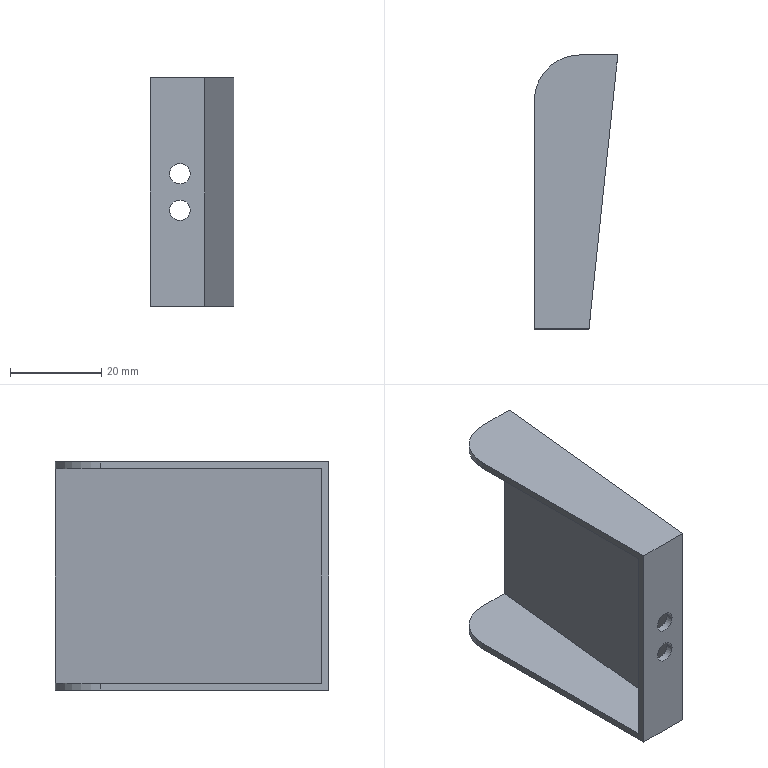Component | SolidWorks | 7.1.02.0001.00.00-0055-1 | 1 solid | 16 faces | box 18.31 x 60 x 50 mm | volume 7614 mm3 | plane 10 | cylinder 6 | commonest cylinder face diameters 4.5 x4 20 x2
STEP:
#1=CARTESIAN_POINT('',(-2.056,1.764,0.1575));
#2=VERTEX_POINT('',#1);
#3=CARTESIAN_POINT('',(-2.233,1.764,0.1575));
#4=VERTEX_POINT('',#3);
#5=CARTESIAN_POINT('',(-2.144,1.764,0.1575));
#6=DIRECTION('',(-0.,-1.,-0.));
#7=DIRECTION('',(-1.,0.,-0.));
#8=AXIS2_PLACEMENT_3D('',#5,#6,#7);
#9=CIRCLE('',#8,0.08858);
#10=EDGE_CURVE('',#2,#4,#9,.T.);
#11=ORIENTED_EDGE('',*,*,#10,.F.);
#12=CARTESIAN_POINT('',(-2.056,1.705,0.1575));
#13=VERTEX_POINT('',#12);
#14=CARTESIAN_POINT('',(-2.056,4.068,0.1575));
#15=DIRECTION('',(0.,-1.,-0.));
#16=VECTOR('',#15,39.37);
#17=LINE('',#14,#16);
#18=EDGE_CURVE('',#2,#13,#17,.T.);
#19=ORIENTED_EDGE('',*,*,#18,.T.);
#20=CARTESIAN_POINT('',(-2.233,1.705,0.1575));
#21=VERTEX_POINT('',#20);
#22=CARTESIAN_POINT('',(-2.144,1.705,0.1575));
#23=DIRECTION('',(0.,-1.,-0.));
#24=DIRECTION('',(-1.,0.,-0.));
#25=AXIS2_PLACEMENT_3D('',#22,#23,#24);
#26=CIRCLE('',#25,0.08858);
#27=EDGE_CURVE('',#13,#21,#26,.T.);
#28=ORIENTED_EDGE('',*,*,#27,.T.);
#29=CARTESIAN_POINT('',(-2.233,4.068,0.1575));
#30=DIRECTION('',(0.,-1.,-0.));
#31=VECTOR('',#30,39.37);
#32=LINE('',#29,#31);
#33=EDGE_CURVE('',#4,#21,#32,.T.);
#34=ORIENTED_EDGE('',*,*,#33,.F.);
#35=EDGE_LOOP('',(#11,#19,#28,#34));
#36=FACE_OUTER_BOUND('',#35,.T.);
#37=CARTESIAN_POINT('',(-2.144,4.068,0.1575));
#38=DIRECTION('',(0.,-1.,-0.));
#39=DIRECTION('',(-1.,0.,-0.));
#40=AXIS2_PLACEMENT_3D('',#37,#38,#39);
#41=CYLINDRICAL_SURFACE('',#40,0.08858);
#42=ADVANCED_FACE('',(#36),#41,.F.);
#43=CARTESIAN_POINT('',(-2.056,1.764,-0.1575));
#44=VERTEX_POINT('',#43);
#45=CARTESIAN_POINT('',(-2.233,1.764,-0.1575));
#46=VERTEX_POINT('',#45);
#47=CARTESIAN_POINT('',(-2.144,1.764,-0.1575));
#48=DIRECTION('',(-0.,-1.,-0.));
#49=DIRECTION('',(-1.,0.,-0.));
#50=AXIS2_PLACEMENT_3D('',#47,#48,#49);
#51=CIRCLE('',#50,0.08858);
#52=EDGE_CURVE('',#44,#46,#51,.T.);
#53=ORIENTED_EDGE('',*,*,#52,.F.);
#54=CARTESIAN_POINT('',(-2.056,1.705,-0.1575));
#55=VERTEX_POINT('',#54);
#56=CARTESIAN_POINT('',(-2.056,4.068,-0.1575));
#57=DIRECTION('',(0.,-1.,-0.));
#58=VECTOR('',#57,39.37);
#59=LINE('',#56,#58);
#60=EDGE_CURVE('',#44,#55,#59,.T.);
#61=ORIENTED_EDGE('',*,*,#60,.T.);
#62=CARTESIAN_POINT('',(-2.233,1.705,-0.1575));
#63=VERTEX_POINT('',#62);
#64=CARTESIAN_POINT('',(-2.144,1.705,-0.1575));
#65=DIRECTION('',(0.,-1.,-0.));
#66=DIRECTION('',(-1.,0.,-0.));
#67=AXIS2_PLACEMENT_3D('',#64,#65,#66);
#68=CIRCLE('',#67,0.08858);
#69=EDGE_CURVE('',#55,#63,#68,.T.);
#70=ORIENTED_EDGE('',*,*,#69,.T.);
#71=CARTESIAN_POINT('',(-2.233,4.068,-0.1575));
#72=DIRECTION('',(0.,-1.,-0.));
#73=VECTOR('',#72,39.37);
#74=LINE('',#71,#73);
#75=EDGE_CURVE('',#46,#63,#74,.T.);
#76=ORIENTED_EDGE('',*,*,#75,.F.);
#77=EDGE_LOOP('',(#53,#61,#70,#76));
#78=FACE_OUTER_BOUND('',#77,.T.);
#79=CARTESIAN_POINT('',(-2.144,4.068,-0.1575));
#80=DIRECTION('',(0.,-1.,-0.));
#81=DIRECTION('',(-1.,0.,-0.));
#82=AXIS2_PLACEMENT_3D('',#79,#80,#81);
#83=CYLINDRICAL_SURFACE('',#82,0.08858);
#84=ADVANCED_FACE('',(#78),#83,.F.);
#85=CARTESIAN_POINT('',(-2.006,4.068,0.9252));
#86=VERTEX_POINT('',#85);
#87=CARTESIAN_POINT('',(-1.739,4.068,0.9252));
#88=VERTEX_POINT('',#87);
#89=CARTESIAN_POINT('',(-2.006,4.068,0.9252));
#90=DIRECTION('',(1.,0.,0.));
#91=VECTOR('',#90,39.37);
#92=LINE('',#89,#91);
#93=EDGE_CURVE('',#86,#88,#92,.T.);
#94=ORIENTED_EDGE('',*,*,#93,.F.);
#95=CARTESIAN_POINT('',(-2.006,4.068,0.9843));
#96=VERTEX_POINT('',#95);
#97=CARTESIAN_POINT('',(-2.006,4.068,-0.9843));
#98=DIRECTION('',(-0.,-0.,1.));
#99=VECTOR('',#98,39.37);
#100=LINE('',#97,#99);
#101=EDGE_CURVE('',#86,#96,#100,.T.);
#102=ORIENTED_EDGE('',*,*,#101,.T.);
#103=CARTESIAN_POINT('',(-1.679,4.068,0.9843));
#104=VERTEX_POINT('',#103);
#105=CARTESIAN_POINT('',(-2.4,4.068,0.9843));
#106=DIRECTION('',(1.,0.,0.));
#107=VECTOR('',#106,39.37);
#108=LINE('',#105,#107);
#109=EDGE_CURVE('',#96,#104,#108,.T.);
#110=ORIENTED_EDGE('',*,*,#109,.T.);
#111=CARTESIAN_POINT('',(-1.679,4.068,-0.9843));
#112=VERTEX_POINT('',#111);
#113=CARTESIAN_POINT('',(-1.679,4.068,-0.9843));
#114=DIRECTION('',(-0.,-0.,1.));
#115=VECTOR('',#114,39.37);
#116=LINE('',#113,#115);
#117=EDGE_CURVE('',#112,#104,#116,.T.);
#118=ORIENTED_EDGE('',*,*,#117,.F.);
#119=CARTESIAN_POINT('',(-2.006,4.068,-0.9843));
#120=VERTEX_POINT('',#119);
#121=CARTESIAN_POINT('',(-2.4,4.068,-0.9843));
#122=DIRECTION('',(1.,0.,0.));
#123=VECTOR('',#122,39.37);
#124=LINE('',#121,#123);
#125=EDGE_CURVE('',#120,#112,#124,.T.);
#126=ORIENTED_EDGE('',*,*,#125,.F.);
#127=CARTESIAN_POINT('',(-2.006,4.068,-0.9252));
#128=VERTEX_POINT('',#127);
#129=CARTESIAN_POINT('',(-2.006,4.068,-0.9843));
#130=DIRECTION('',(-0.,-0.,1.));
#131=VECTOR('',#130,39.37);
#132=LINE('',#129,#131);
#133=EDGE_CURVE('',#120,#128,#132,.T.);
#134=ORIENTED_EDGE('',*,*,#133,.T.);
#135=CARTESIAN_POINT('',(-1.739,4.068,-0.9252));
#136=VERTEX_POINT('',#135);
#137=CARTESIAN_POINT('',(-2.006,4.068,-0.9252));
#138=DIRECTION('',(1.,0.,0.));
#139=VECTOR('',#138,39.37);
#140=LINE('',#137,#139);
#141=EDGE_CURVE('',#128,#136,#140,.T.);
#142=ORIENTED_EDGE('',*,*,#141,.T.);
#143=CARTESIAN_POINT('',(-1.739,4.068,0.9252));
#144=DIRECTION('',(0.,0.,-1.));
#145=VECTOR('',#144,39.37);
#146=LINE('',#143,#145);
#147=EDGE_CURVE('',#88,#136,#146,.T.);
#148=ORIENTED_EDGE('',*,*,#147,.F.);
#149=EDGE_LOOP('',(#94,#102,#110,#118,#126,#134,#142,#148));
#150=FACE_OUTER_BOUND('',#149,.T.);
#151=CARTESIAN_POINT('',(-2.4,4.068,-0.9843));
#152=DIRECTION('',(0.,-1.,-0.));
#153=DIRECTION('',(-1.,-0.,-0.));
#154=AXIS2_PLACEMENT_3D('',#151,#152,#153);
#155=PLANE('',#154);
#156=ADVANCED_FACE('',(#150),#155,.F.);
#157=CARTESIAN_POINT('',(-2.4,1.764,0.9252));
#158=VERTEX_POINT('',#157);
#159=CARTESIAN_POINT('',(-2.4,3.674,0.9252));
#160=VERTEX_POINT('',#159);
#161=CARTESIAN_POINT('',(-2.4,1.764,0.9252));
#162=DIRECTION('',(-0.,1.,0.));
#163=VECTOR('',#162,39.37);
#164=LINE('',#161,#163);
#165=EDGE_CURVE('',#158,#160,#164,.T.);
#166=ORIENTED_EDGE('',*,*,#165,.F.);
#167=CARTESIAN_POINT('',(-2.4,1.764,-0.9252));
#168=VERTEX_POINT('',#167);
#169=CARTESIAN_POINT('',(-2.4,1.764,0.9252));
#170=DIRECTION('',(0.,0.,-1.));
#171=VECTOR('',#170,39.37);
#172=LINE('',#169,#171);
#173=EDGE_CURVE('',#158,#168,#172,.T.);
#174=ORIENTED_EDGE('',*,*,#173,.T.);
#175=CARTESIAN_POINT('',(-2.4,3.674,-0.9252));
#176=VERTEX_POINT('',#175);
#177=CARTESIAN_POINT('',(-2.4,1.764,-0.9252));
#178=DIRECTION('',(-0.,1.,0.));
#179=VECTOR('',#178,39.37);
#180=LINE('',#177,#179);
#181=EDGE_CURVE('',#168,#176,#180,.T.);
#182=ORIENTED_EDGE('',*,*,#181,.T.);
#183=CARTESIAN_POINT('',(-2.4,3.674,-0.9843));
#184=VERTEX_POINT('',#183);
#185=CARTESIAN_POINT('',(-2.4,3.674,-0.9843));
#186=DIRECTION('',(0.,0.,-1.));
#187=VECTOR('',#186,39.37);
#188=LINE('',#185,#187);
#189=EDGE_CURVE('',#176,#184,#188,.T.);
#190=ORIENTED_EDGE('',*,*,#189,.T.);
#191=CARTESIAN_POINT('',(-2.4,1.705,-0.9843));
#192=VERTEX_POINT('',#191);
#193=CARTESIAN_POINT('',(-2.4,4.068,-0.9843));
#194=DIRECTION('',(-0.,1.,0.));
#195=VECTOR('',#194,39.37);
#196=LINE('',#193,#195);
#197=EDGE_CURVE('',#192,#184,#196,.T.);
#198=ORIENTED_EDGE('',*,*,#197,.F.);
#199=CARTESIAN_POINT('',(-2.4,1.705,0.9843));
#200=VERTEX_POINT('',#199);
#201=CARTESIAN_POINT('',(-2.4,1.705,-0.9843));
#202=DIRECTION('',(-0.,-0.,1.));
#203=VECTOR('',#202,39.37);
#204=LINE('',#201,#203);
#205=EDGE_CURVE('',#192,#200,#204,.T.);
#206=ORIENTED_EDGE('',*,*,#205,.T.);
#207=CARTESIAN_POINT('',(-2.4,3.674,0.9843));
#208=VERTEX_POINT('',#207);
#209=CARTESIAN_POINT('',(-2.4,4.068,0.9843));
#210=DIRECTION('',(-0.,1.,0.));
#211=VECTOR('',#210,39.37);
#212=LINE('',#209,#211);
#213=EDGE_CURVE('',#200,#208,#212,.T.);
#214=ORIENTED_EDGE('',*,*,#213,.T.);
#215=CARTESIAN_POINT('',(-2.4,3.674,-0.9843));
#216=DIRECTION('',(0.,0.,-1.));
#217=VECTOR('',#216,39.37);
#218=LINE('',#215,#217);
#219=EDGE_CURVE('',#208,#160,#218,.T.);
#220=ORIENTED_EDGE('',*,*,#219,.T.);
#221=EDGE_LOOP('',(#166,#174,#182,#190,#198,#206,#214,#220));
#222=FACE_OUTER_BOUND('',#221,.T.);
#223=CARTESIAN_POINT('',(-2.4,4.068,-0.9843));
#224=DIRECTION('',(1.,0.,0.));
#225=DIRECTION('',(-0.,-0.,1.));
#226=AXIS2_PLACEMENT_3D('',#223,#224,#225);
#227=PLANE('',#226);
#228=ADVANCED_FACE('',(#222),#227,.F.);
#229=ORIENTED_EDGE('',*,*,#101,.F.);
#230=CARTESIAN_POINT('',(-2.006,3.674,0.9252));
#231=DIRECTION('',(0.,0.,-1.));
#232=DIRECTION('',(0.,-1.,0.));
#233=AXIS2_PLACEMENT_3D('',#230,#231,#232);
#234=CIRCLE('',#233,0.3937);
#235=EDGE_CURVE('',#160,#86,#234,.T.);
#236=ORIENTED_EDGE('',*,*,#235,.F.);
#237=ORIENTED_EDGE('',*,*,#219,.F.);
#238=CARTESIAN_POINT('',(-2.006,3.674,0.9843));
#239=DIRECTION('',(-0.,-0.,1.));
#240=DIRECTION('',(0.,-1.,0.));
#241=AXIS2_PLACEMENT_3D('',#238,#239,#240);
#242=CIRCLE('',#241,0.3937);
#243=EDGE_CURVE('',#96,#208,#242,.T.);
#244=ORIENTED_EDGE('',*,*,#243,.F.);
#245=EDGE_LOOP('',(#229,#236,#237,#244));
#246=FACE_OUTER_BOUND('',#245,.T.);
#247=CARTESIAN_POINT('',(-2.006,3.674,-0.9843));
#248=DIRECTION('',(-0.,-0.,1.));
#249=DIRECTION('',(0.,1.,0.));
#250=AXIS2_PLACEMENT_3D('',#247,#248,#249);
#251=CYLINDRICAL_SURFACE('',#250,0.3937);
#252=ADVANCED_FACE('',(#246),#251,.T.);
#253=CARTESIAN_POINT('',(-1.928,1.705,0.9843));
#254=VERTEX_POINT('',#253);
#255=CARTESIAN_POINT('',(-1.928,1.705,0.9843));
#256=DIRECTION('',(-0.1045,-0.9945,-0.));
#257=VECTOR('',#256,39.37);
#258=LINE('',#255,#257);
#259=EDGE_CURVE('',#104,#254,#258,.T.);
#260=ORIENTED_EDGE('',*,*,#259,.T.);
#261=CARTESIAN_POINT('',(-1.928,1.705,-0.9843));
#262=VERTEX_POINT('',#261);
#263=CARTESIAN_POINT('',(-1.928,1.705,-0.9843));
#264=DIRECTION('',(-0.,-0.,1.));
#265=VECTOR('',#264,39.37);
#266=LINE('',#263,#265);
#267=EDGE_CURVE('',#262,#254,#266,.T.);
#268=ORIENTED_EDGE('',*,*,#267,.F.);
#269=CARTESIAN_POINT('',(-1.928,1.705,-0.9843));
#270=DIRECTION('',(-0.1045,-0.9945,-0.));
#271=VECTOR('',#270,39.37);
#272=LINE('',#269,#271);
#273=EDGE_CURVE('',#112,#262,#272,.T.);
#274=ORIENTED_EDGE('',*,*,#273,.F.);
#275=ORIENTED_EDGE('',*,*,#117,.T.);
#276=EDGE_LOOP('',(#260,#268,#274,#275));
#277=FACE_OUTER_BOUND('',#276,.T.);
#278=CARTESIAN_POINT('',(-1.928,1.705,-0.9843));
#279=DIRECTION('',(-0.9945,0.1045,-0.));
#280=DIRECTION('',(0.1045,0.9945,0.));
#281=AXIS2_PLACEMENT_3D('',#278,#279,#280);
#282=PLANE('',#281);
#283=ADVANCED_FACE('',(#277),#282,.F.);
#284=CARTESIAN_POINT('',(-2.144,1.705,0.1575));
#285=DIRECTION('',(0.,-1.,-0.));
#286=DIRECTION('',(-1.,0.,-0.));
#287=AXIS2_PLACEMENT_3D('',#284,#285,#286);
#288=CIRCLE('',#287,0.08858);
#289=EDGE_CURVE('',#21,#13,#288,.T.);
#290=ORIENTED_EDGE('',*,*,#289,.F.);
#291=ORIENTED_EDGE('',*,*,#27,.F.);
#292=EDGE_LOOP('',(#290,#291));
#293=FACE_BOUND('',#292,.T.);
#294=CARTESIAN_POINT('',(-2.144,1.705,-0.1575));
#295=DIRECTION('',(0.,-1.,-0.));
#296=DIRECTION('',(-1.,0.,-0.));
#297=AXIS2_PLACEMENT_3D('',#294,#295,#296);
#298=CIRCLE('',#297,0.08858);
#299=EDGE_CURVE('',#63,#55,#298,.T.);
#300=ORIENTED_EDGE('',*,*,#299,.F.);
#301=ORIENTED_EDGE('',*,*,#69,.F.);
#302=EDGE_LOOP('',(#300,#301));
#303=FACE_BOUND('',#302,.T.);
#304=CARTESIAN_POINT('',(-2.4,1.705,0.9843));
#305=DIRECTION('',(-1.,0.,-0.));
#306=VECTOR('',#305,39.37);
#307=LINE('',#304,#306);
#308=EDGE_CURVE('',#254,#200,#307,.T.);
#309=ORIENTED_EDGE('',*,*,#308,.T.);
#310=ORIENTED_EDGE('',*,*,#205,.F.);
#311=CARTESIAN_POINT('',(-2.4,1.705,-0.9843));
#312=DIRECTION('',(-1.,0.,-0.));
#313=VECTOR('',#312,39.37);
#314=LINE('',#311,#313);
#315=EDGE_CURVE('',#262,#192,#314,.T.);
#316=ORIENTED_EDGE('',*,*,#315,.F.);
#317=ORIENTED_EDGE('',*,*,#267,.T.);
#318=EDGE_LOOP('',(#309,#310,#316,#317));
#319=FACE_OUTER_BOUND('',#318,.T.);
#320=CARTESIAN_POINT('',(-2.4,1.705,-0.9843));
#321=DIRECTION('',(0.,1.,0.));
#322=DIRECTION('',(1.,-0.,0.));
#323=AXIS2_PLACEMENT_3D('',#320,#321,#322);
#324=PLANE('',#323);
#325=ADVANCED_FACE('',(#293,#303,#319),#324,.F.);
#326=ORIENTED_EDGE('',*,*,#197,.T.);
#327=CARTESIAN_POINT('',(-2.006,3.674,-0.9843));
#328=DIRECTION('',(0.,0.,-1.));
#329=DIRECTION('',(0.,-1.,0.));
#330=AXIS2_PLACEMENT_3D('',#327,#328,#329);
#331=CIRCLE('',#330,0.3937);
#332=EDGE_CURVE('',#184,#120,#331,.T.);
#333=ORIENTED_EDGE('',*,*,#332,.T.);
#334=ORIENTED_EDGE('',*,*,#125,.T.);
#335=ORIENTED_EDGE('',*,*,#273,.T.);
#336=ORIENTED_EDGE('',*,*,#315,.T.);
#337=EDGE_LOOP('',(#326,#333,#334,#335,#336));
#338=FACE_OUTER_BOUND('',#337,.T.);
#339=CARTESIAN_POINT('',(-2.203,2.886,-0.9843));
#340=DIRECTION('',(0.,0.,-1.));
#341=DIRECTION('',(0.,-1.,-0.));
#342=AXIS2_PLACEMENT_3D('',#339,#340,#341);
#343=PLANE('',#342);
#344=ADVANCED_FACE('',(#338),#343,.T.);
#345=ORIENTED_EDGE('',*,*,#109,.F.);
#346=ORIENTED_EDGE('',*,*,#243,.T.);
#347=ORIENTED_EDGE('',*,*,#213,.F.);
#348=ORIENTED_EDGE('',*,*,#308,.F.);
#349=ORIENTED_EDGE('',*,*,#259,.F.);
#350=EDGE_LOOP('',(#345,#346,#347,#348,#349));
#351=FACE_OUTER_BOUND('',#350,.T.);
#352=CARTESIAN_POINT('',(-2.203,2.886,0.9843));
#353=DIRECTION('',(0.,0.,-1.));
#354=DIRECTION('',(0.,-1.,-0.));
#355=AXIS2_PLACEMENT_3D('',#352,#353,#354);
#356=PLANE('',#355);
#357=ADVANCED_FACE('',(#351),#356,.F.);
#358=CARTESIAN_POINT('',(-2.006,3.674,-0.9252));
#359=DIRECTION('',(0.,0.,-1.));
#360=DIRECTION('',(0.,-1.,0.));
#361=AXIS2_PLACEMENT_3D('',#358,#359,#360);
#362=CIRCLE('',#361,0.3937);
#363=EDGE_CURVE('',#176,#128,#362,.T.);
#364=ORIENTED_EDGE('',*,*,#363,.T.);
#365=ORIENTED_EDGE('',*,*,#133,.F.);
#366=ORIENTED_EDGE('',*,*,#332,.F.);
#367=ORIENTED_EDGE('',*,*,#189,.F.);
#368=EDGE_LOOP('',(#364,#365,#366,#367));
#369=FACE_OUTER_BOUND('',#368,.T.);
#370=CARTESIAN_POINT('',(-2.006,3.674,-0.9843));
#371=DIRECTION('',(-0.,-0.,1.));
#372=DIRECTION('',(0.,1.,0.));
#373=AXIS2_PLACEMENT_3D('',#370,#371,#372);
#374=CYLINDRICAL_SURFACE('',#373,0.3937);
#375=ADVANCED_FACE('',(#369),#374,.T.);
#376=CARTESIAN_POINT('',(-2.144,1.764,0.1575));
#377=DIRECTION('',(-0.,-1.,-0.));
#378=DIRECTION('',(-1.,0.,-0.));
#379=AXIS2_PLACEMENT_3D('',#376,#377,#378);
#380=CIRCLE('',#379,0.08858);
#381=EDGE_CURVE('',#4,#2,#380,.T.);
#382=ORIENTED_EDGE('',*,*,#381,.T.);
#383=ORIENTED_EDGE('',*,*,#10,.T.);
#384=EDGE_LOOP('',(#382,#383));
#385=FACE_BOUND('',#384,.T.);
#386=CARTESIAN_POINT('',(-2.144,1.764,-0.1575));
#387=DIRECTION('',(-0.,-1.,-0.));
#388=DIRECTION('',(-1.,0.,-0.));
#389=AXIS2_PLACEMENT_3D('',#386,#387,#388);
#390=CIRCLE('',#389,0.08858);
#391=EDGE_CURVE('',#46,#44,#390,.T.);
#392=ORIENTED_EDGE('',*,*,#391,.T.);
#393=ORIENTED_EDGE('',*,*,#52,.T.);
#394=EDGE_LOOP('',(#392,#393));
#395=FACE_BOUND('',#394,.T.);
#396=CARTESIAN_POINT('',(-1.981,1.764,-0.9252));
#397=VERTEX_POINT('',#396);
#398=CARTESIAN_POINT('',(-1.981,1.764,-0.9252));
#399=DIRECTION('',(-1.,0.,-0.));
#400=VECTOR('',#399,39.37);
#401=LINE('',#398,#400);
#402=EDGE_CURVE('',#397,#168,#401,.T.);
#403=ORIENTED_EDGE('',*,*,#402,.T.);
#404=ORIENTED_EDGE('',*,*,#173,.F.);
#405=CARTESIAN_POINT('',(-1.981,1.764,0.9252));
#406=VERTEX_POINT('',#405);
#407=CARTESIAN_POINT('',(-1.981,1.764,0.9252));
#408=DIRECTION('',(-1.,0.,-0.));
#409=VECTOR('',#408,39.37);
#410=LINE('',#407,#409);
#411=EDGE_CURVE('',#406,#158,#410,.T.);
#412=ORIENTED_EDGE('',*,*,#411,.F.);
#413=CARTESIAN_POINT('',(-1.981,1.764,0.9252));
#414=DIRECTION('',(0.,0.,-1.));
#415=VECTOR('',#414,39.37);
#416=LINE('',#413,#415);
#417=EDGE_CURVE('',#406,#397,#416,.T.);
#418=ORIENTED_EDGE('',*,*,#417,.T.);
#419=EDGE_LOOP('',(#403,#404,#412,#418));
#420=FACE_OUTER_BOUND('',#419,.T.);
#421=CARTESIAN_POINT('',(-1.981,1.764,0.9252));
#422=DIRECTION('',(-0.,-1.,-0.));
#423=DIRECTION('',(-1.,0.,-0.));
#424=AXIS2_PLACEMENT_3D('',#421,#422,#423);
#425=PLANE('',#424);
#426=ADVANCED_FACE('',(#385,#395,#420),#425,.F.);
#427=CARTESIAN_POINT('',(-1.739,4.068,-0.9252));
#428=DIRECTION('',(-0.1045,-0.9945,-0.));
#429=VECTOR('',#428,39.37);
#430=LINE('',#427,#429);
#431=EDGE_CURVE('',#136,#397,#430,.T.);
#432=ORIENTED_EDGE('',*,*,#431,.T.);
#433=ORIENTED_EDGE('',*,*,#417,.F.);
#434=CARTESIAN_POINT('',(-1.739,4.068,0.9252));
#435=DIRECTION('',(-0.1045,-0.9945,-0.));
#436=VECTOR('',#435,39.37);
#437=LINE('',#434,#436);
#438=EDGE_CURVE('',#88,#406,#437,.T.);
#439=ORIENTED_EDGE('',*,*,#438,.F.);
#440=ORIENTED_EDGE('',*,*,#147,.T.);
#441=EDGE_LOOP('',(#432,#433,#439,#440));
#442=FACE_OUTER_BOUND('',#441,.T.);
#443=CARTESIAN_POINT('',(-1.739,4.068,0.9252));
#444=DIRECTION('',(0.9945,-0.1045,0.));
#445=DIRECTION('',(-0.1045,-0.9945,-0.));
#446=AXIS2_PLACEMENT_3D('',#443,#444,#445);
#447=PLANE('',#446);
#448=ADVANCED_FACE('',(#442),#447,.F.);
#449=ORIENTED_EDGE('',*,*,#235,.T.);
#450=ORIENTED_EDGE('',*,*,#93,.T.);
#451=ORIENTED_EDGE('',*,*,#438,.T.);
#452=ORIENTED_EDGE('',*,*,#411,.T.);
#453=ORIENTED_EDGE('',*,*,#165,.T.);
#454=EDGE_LOOP('',(#449,#450,#451,#452,#453));
#455=FACE_OUTER_BOUND('',#454,.T.);
#456=CARTESIAN_POINT('',(-2.006,3.674,0.9252));
#457=DIRECTION('',(0.,0.,-1.));
#458=DIRECTION('',(0.,-1.,-0.));
#459=AXIS2_PLACEMENT_3D('',#456,#457,#458);
#460=PLANE('',#459);
#461=ADVANCED_FACE('',(#455),#460,.T.);
#462=ORIENTED_EDGE('',*,*,#363,.F.);
#463=ORIENTED_EDGE('',*,*,#181,.F.);
#464=ORIENTED_EDGE('',*,*,#402,.F.);
#465=ORIENTED_EDGE('',*,*,#431,.F.);
#466=ORIENTED_EDGE('',*,*,#141,.F.);
#467=EDGE_LOOP('',(#462,#463,#464,#465,#466));
#468=FACE_OUTER_BOUND('',#467,.T.);
#469=CARTESIAN_POINT('',(-2.006,3.674,-0.9252));
#470=DIRECTION('',(0.,0.,-1.));
#471=DIRECTION('',(0.,-1.,-0.));
#472=AXIS2_PLACEMENT_3D('',#469,#470,#471);
#473=PLANE('',#472);
#474=ADVANCED_FACE('',(#468),#473,.F.);
#475=ORIENTED_EDGE('',*,*,#60,.F.);
#476=ORIENTED_EDGE('',*,*,#391,.F.);
#477=ORIENTED_EDGE('',*,*,#75,.T.);
#478=ORIENTED_EDGE('',*,*,#299,.T.);
#479=EDGE_LOOP('',(#475,#476,#477,#478));
#480=FACE_OUTER_BOUND('',#479,.T.);
#481=CARTESIAN_POINT('',(-2.144,4.068,-0.1575));
#482=DIRECTION('',(0.,-1.,-0.));
#483=DIRECTION('',(-1.,0.,-0.));
#484=AXIS2_PLACEMENT_3D('',#481,#482,#483);
#485=CYLINDRICAL_SURFACE('',#484,0.08858);
#486=ADVANCED_FACE('',(#480),#485,.F.);
#487=ORIENTED_EDGE('',*,*,#18,.F.);
#488=ORIENTED_EDGE('',*,*,#381,.F.);
#489=ORIENTED_EDGE('',*,*,#33,.T.);
#490=ORIENTED_EDGE('',*,*,#289,.T.);
#491=EDGE_LOOP('',(#487,#488,#489,#490));
#492=FACE_OUTER_BOUND('',#491,.T.);
#493=CARTESIAN_POINT('',(-2.144,4.068,0.1575));
#494=DIRECTION('',(0.,-1.,-0.));
#495=DIRECTION('',(-1.,0.,-0.));
#496=AXIS2_PLACEMENT_3D('',#493,#494,#495);
#497=CYLINDRICAL_SURFACE('',#496,0.08858);
#498=ADVANCED_FACE('',(#492),#497,.F.);
#499=CLOSED_SHELL('',(#42,#84,#156,#228,#252,#283,#325,#344,#357,#375,#426,#448,#461,#474,#486,#498));
#500=MANIFOLD_SOLID_BREP('',#499);
#501=CARTESIAN_POINT('',(0.,0.,0.));
#502=DIRECTION('',(0.,0.,1.));
#503=DIRECTION('',(1.,0.,0.));
#504=AXIS2_PLACEMENT_3D('',#501,#502,#503);
#505=(LENGTH_UNIT()NAMED_UNIT(*)SI_UNIT($,.METRE.));
#506=LENGTH_MEASURE_WITH_UNIT(LENGTH_MEASURE(0.0254),#505);
#507=DIMENSIONAL_EXPONENTS(1.,0.,0.,0.,0.,0.,0.);
#508=(CONVERSION_BASED_UNIT('',#506)LENGTH_UNIT()NAMED_UNIT(#507));
#509=UNCERTAINTY_MEASURE_WITH_UNIT(LENGTH_MEASURE(0.00001),#508,'','');
#510=(NAMED_UNIT(*)PLANE_ANGLE_UNIT()SI_UNIT($,.RADIAN.));
#511=(NAMED_UNIT(*)SI_UNIT($,.STERADIAN.)SOLID_ANGLE_UNIT());
#512=(GEOMETRIC_REPRESENTATION_CONTEXT(3)GLOBAL_UNCERTAINTY_ASSIGNED_CONTEXT((#509))GLOBAL_UNIT_ASSIGNED_CONTEXT((#508,#510,#511))REPRESENTATION_CONTEXT('',''));
#513=ADVANCED_BREP_SHAPE_REPRESENTATION('',(#500,#504),#512);
#514=COLOUR_RGB('',0.7922,0.8196,0.9333);
#515=FILL_AREA_STYLE_COLOUR('',#514);
#516=FILL_AREA_STYLE('',(#515));
#517=SURFACE_STYLE_FILL_AREA(#516);
#518=SURFACE_SIDE_STYLE('',(#517));
#519=SURFACE_STYLE_USAGE(.BOTH.,#518);
#520=PRESENTATION_STYLE_ASSIGNMENT((#519));
#521=STYLED_ITEM('',(#520),#500);
#522=(LENGTH_UNIT()NAMED_UNIT(*)SI_UNIT($,.METRE.));
#523=LENGTH_MEASURE_WITH_UNIT(LENGTH_MEASURE(0.0254),#522);
#524=DIMENSIONAL_EXPONENTS(1.,0.,0.,0.,0.,0.,0.);
#525=(CONVERSION_BASED_UNIT('',#523)LENGTH_UNIT()NAMED_UNIT(#524));
#526=UNCERTAINTY_MEASURE_WITH_UNIT(LENGTH_MEASURE(0.00001),#525,'','');
#527=(NAMED_UNIT(*)PLANE_ANGLE_UNIT()SI_UNIT($,.RADIAN.));
#528=(NAMED_UNIT(*)SI_UNIT($,.STERADIAN.)SOLID_ANGLE_UNIT());
#529=(GEOMETRIC_REPRESENTATION_CONTEXT(3)GLOBAL_UNCERTAINTY_ASSIGNED_CONTEXT((#526))GLOBAL_UNIT_ASSIGNED_CONTEXT((#525,#527,#528))REPRESENTATION_CONTEXT('',''));
#530=MECHANICAL_DESIGN_GEOMETRIC_PRESENTATION_REPRESENTATION('',(#521),#529);
#531=PRESENTATION_LAYER_ASSIGNMENT('','',(#521));